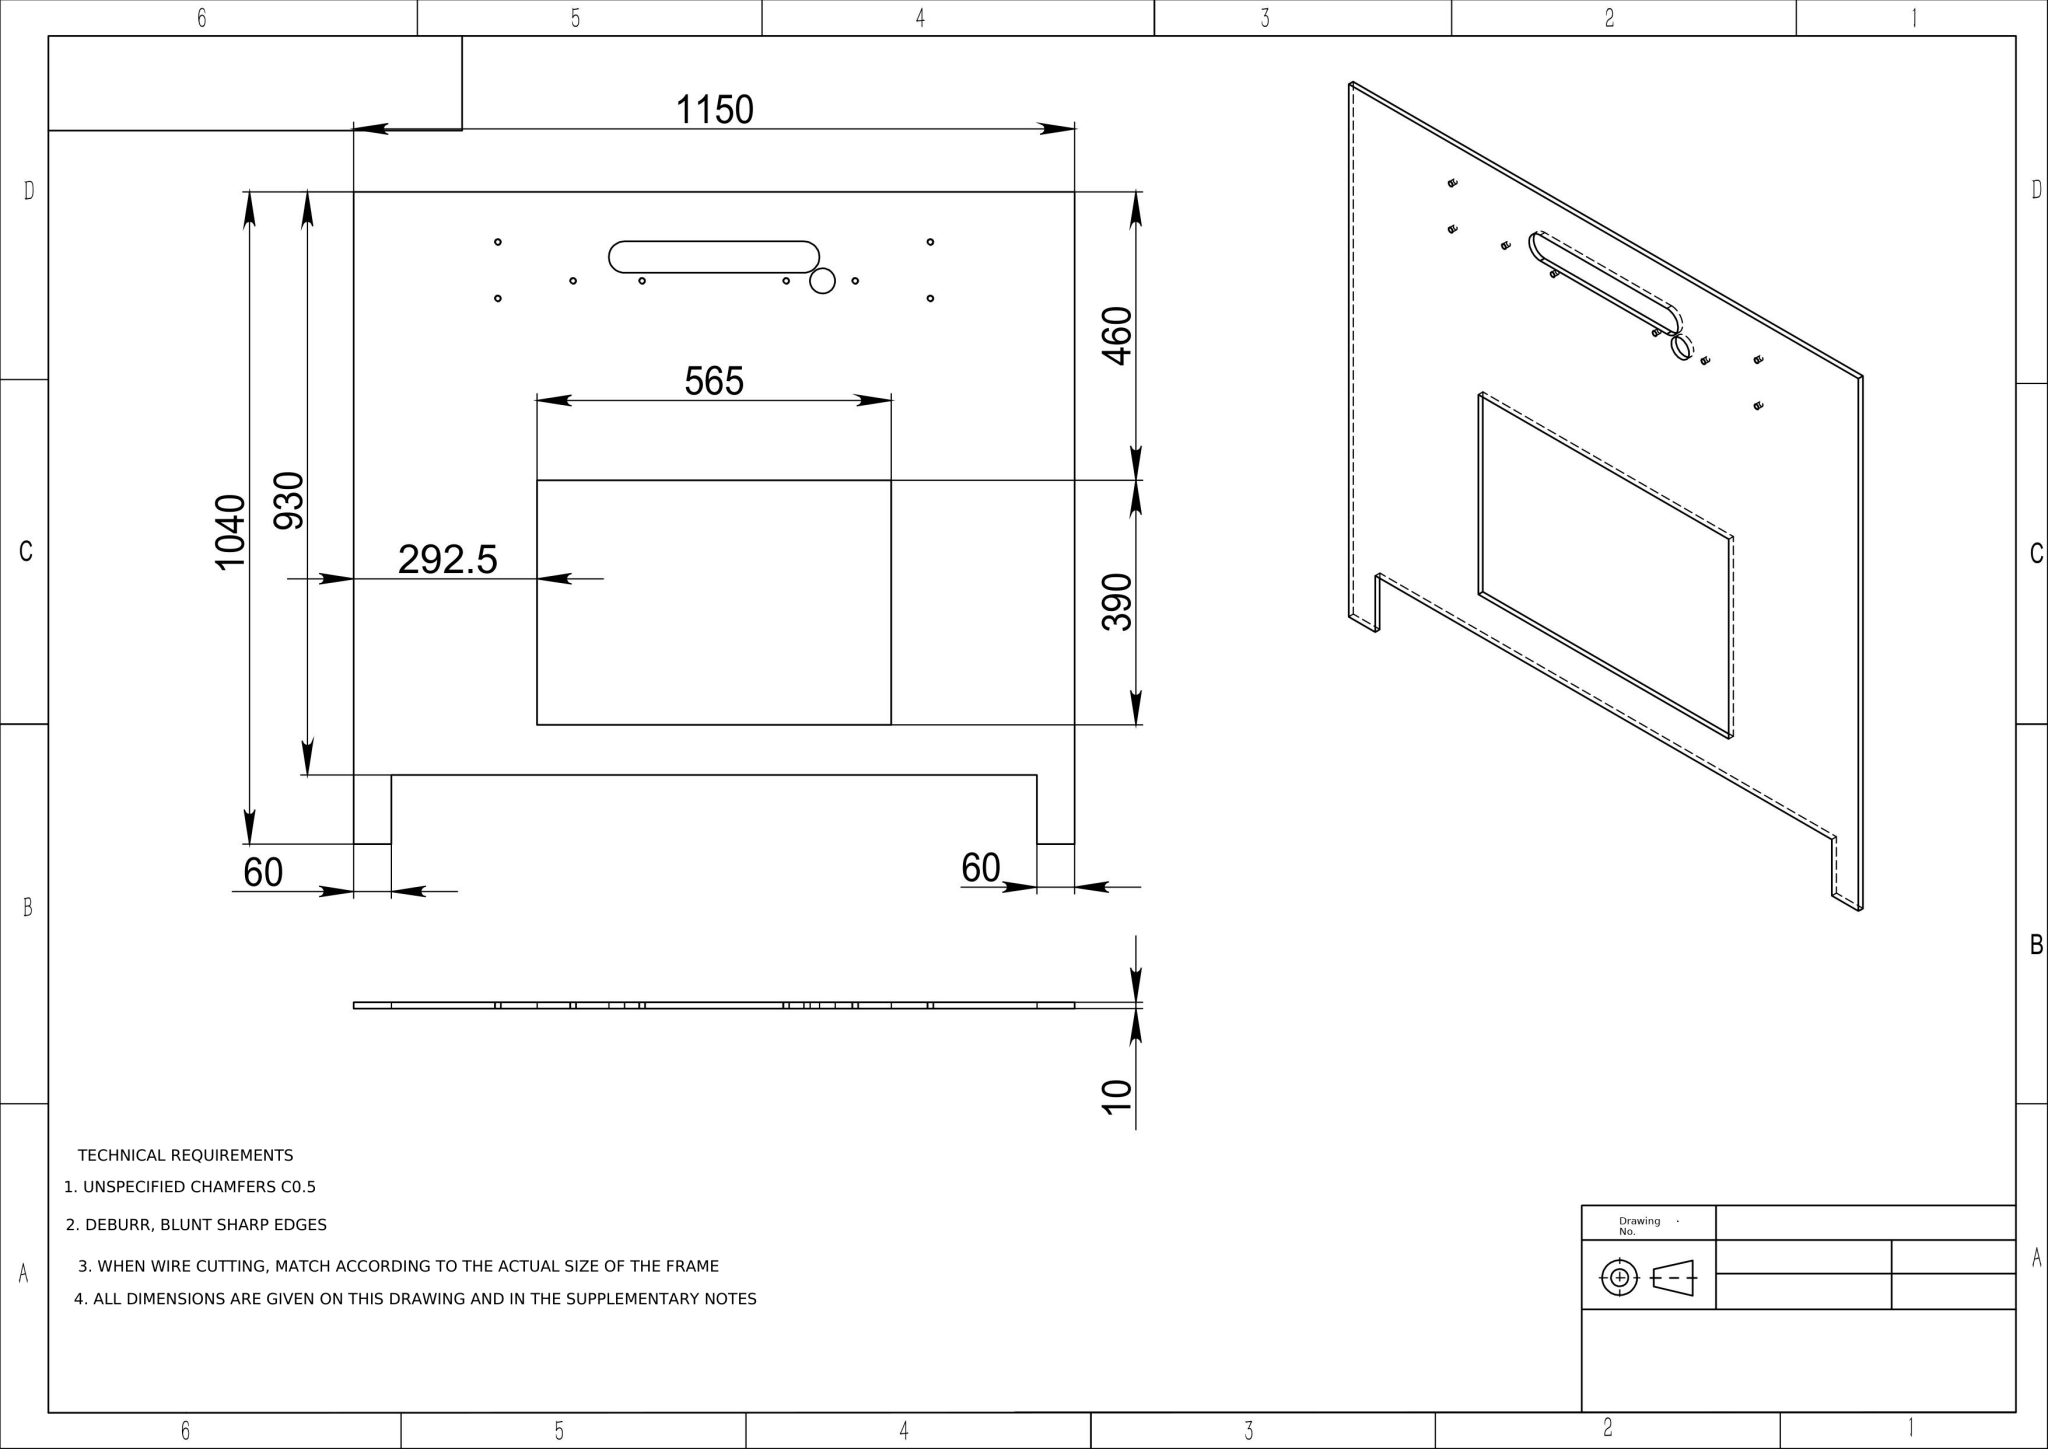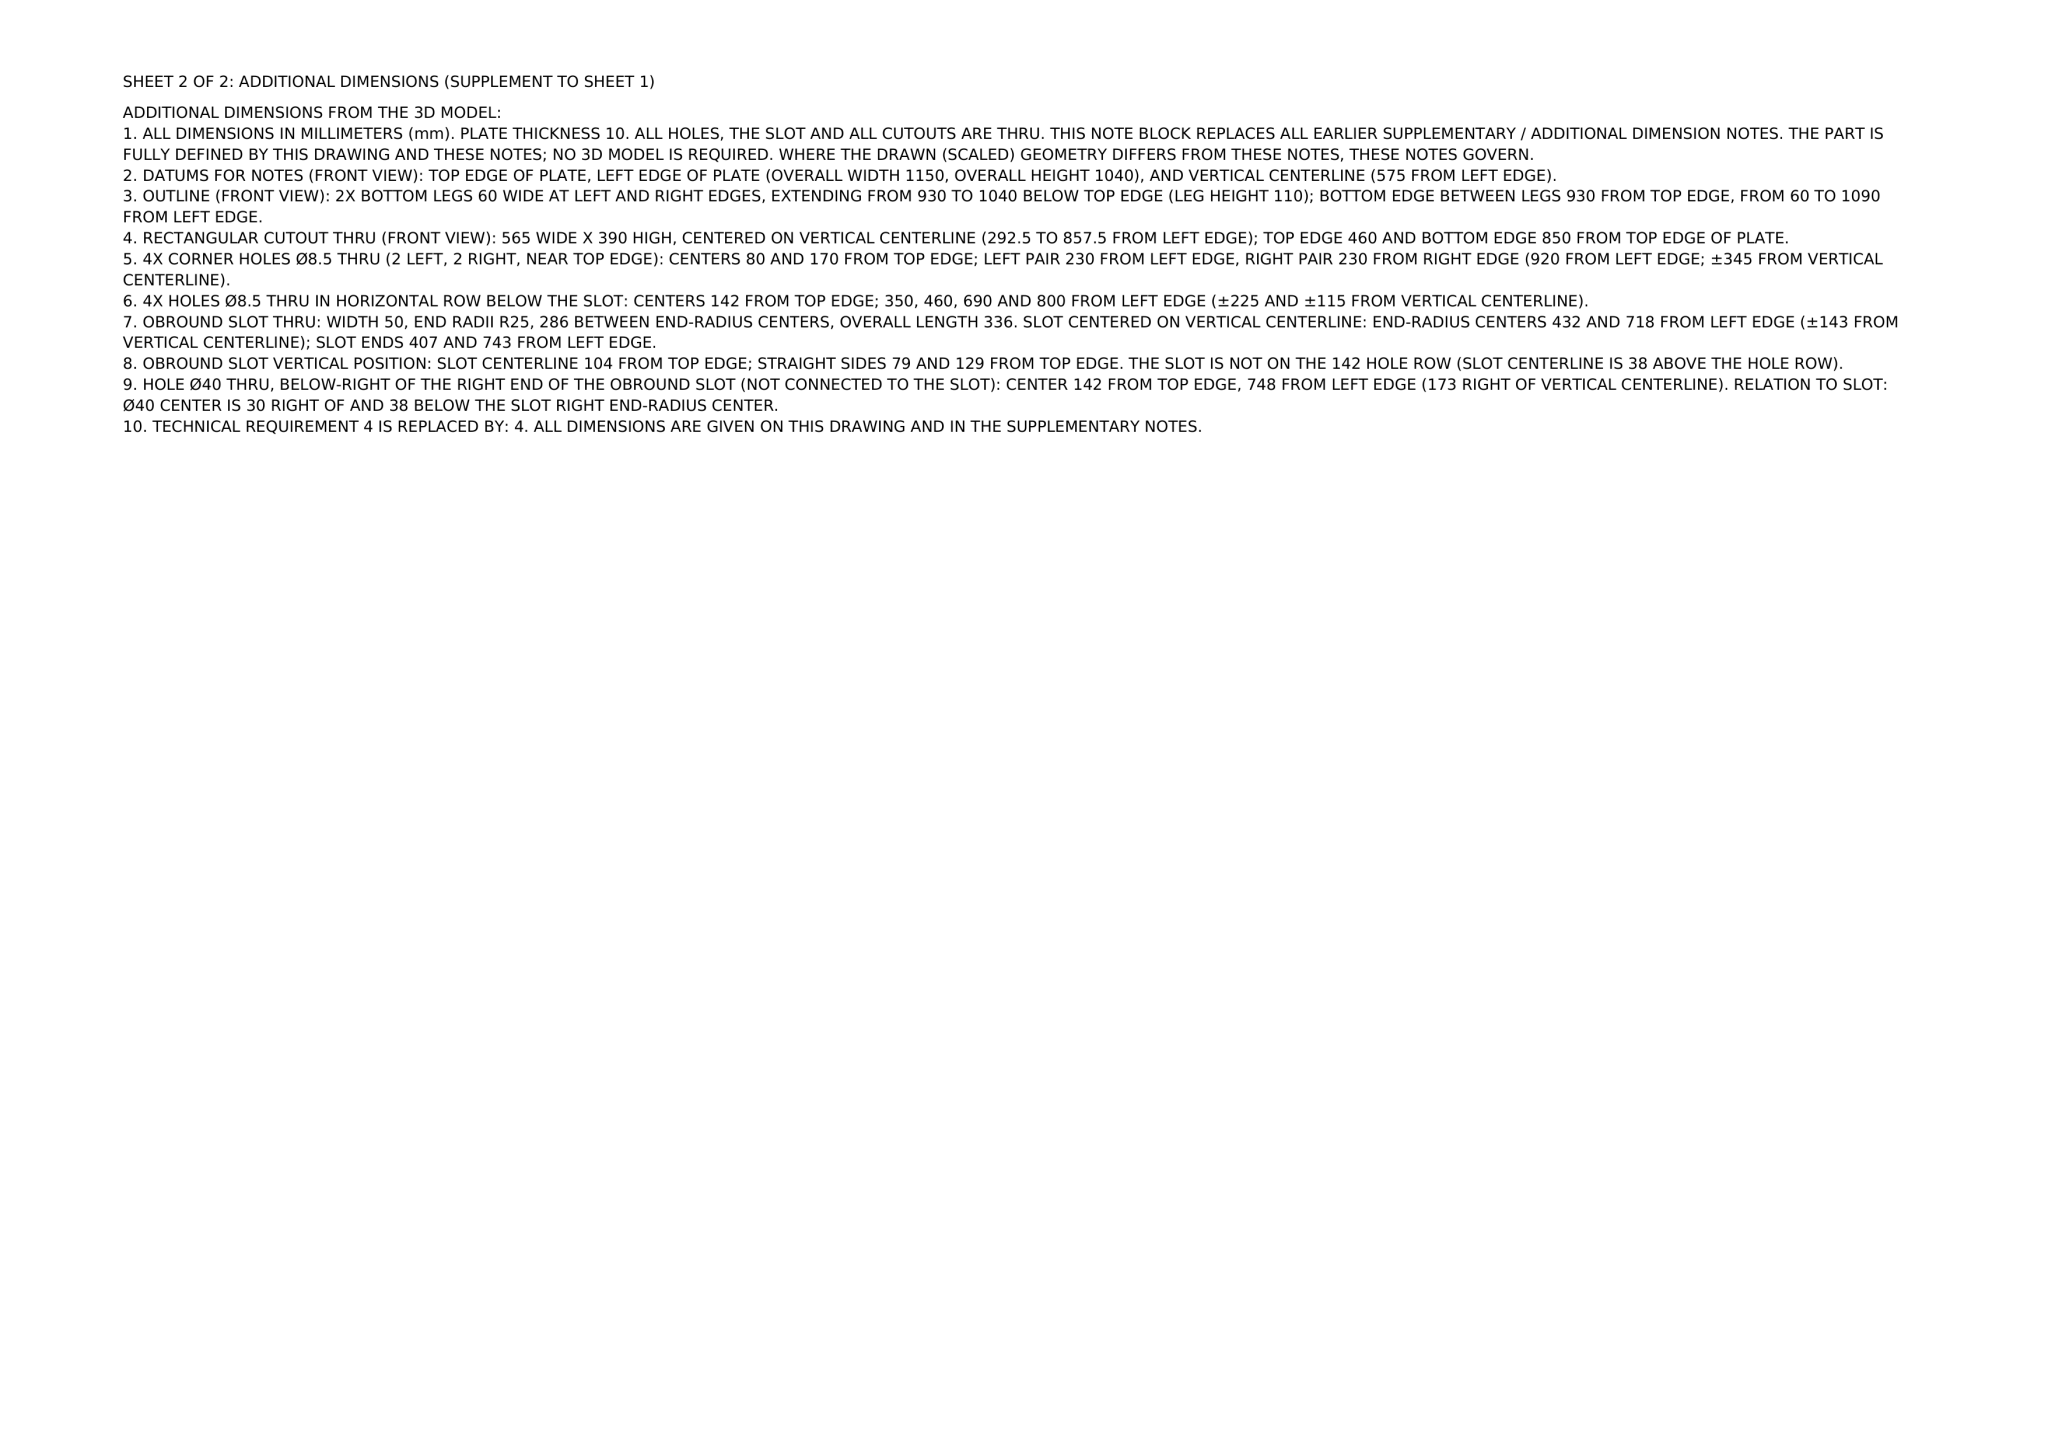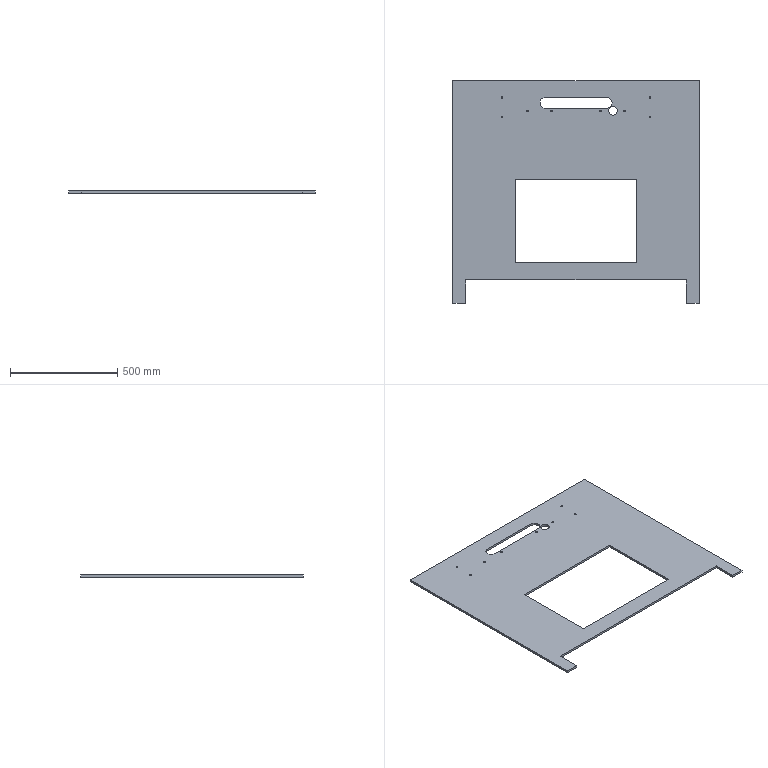Part | NX | mm | 1 solid | 37 faces | box 1150 x 1040 x 10 mm | volume 8443759 mm3 | cylinder 21 | plane 16 | commonest cylinder face diameters 8.5 x16 50 x3 40 x2